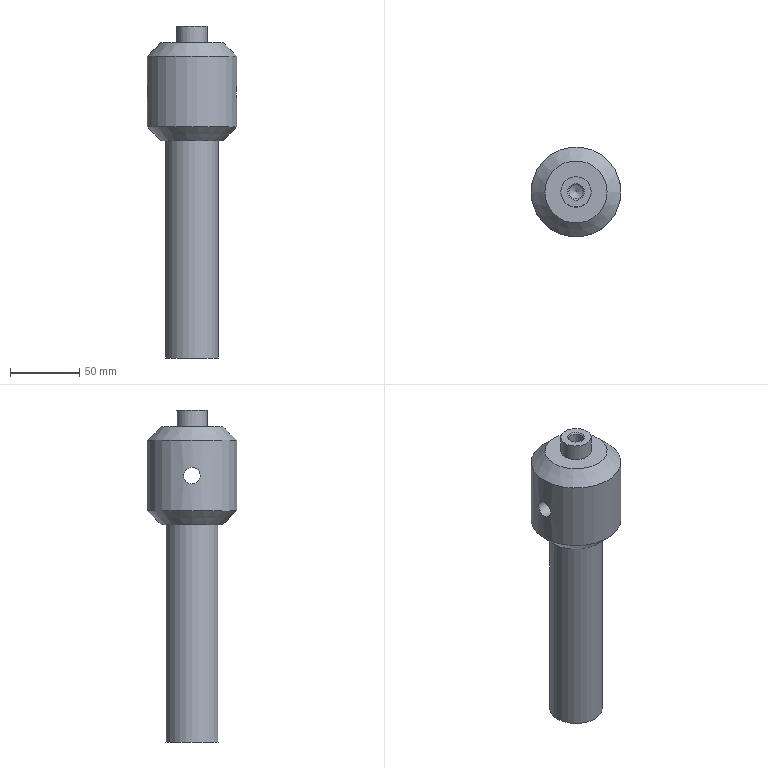Component | NX | SCREW_SPINDLE | 1 solid | 13 faces | volume 389563 mm3 | cylinder 5 | plane 4 | cone 4 | commonest cylinder face diameters 65 x1 38 x1 22 x1 12 x1 10.3 x1